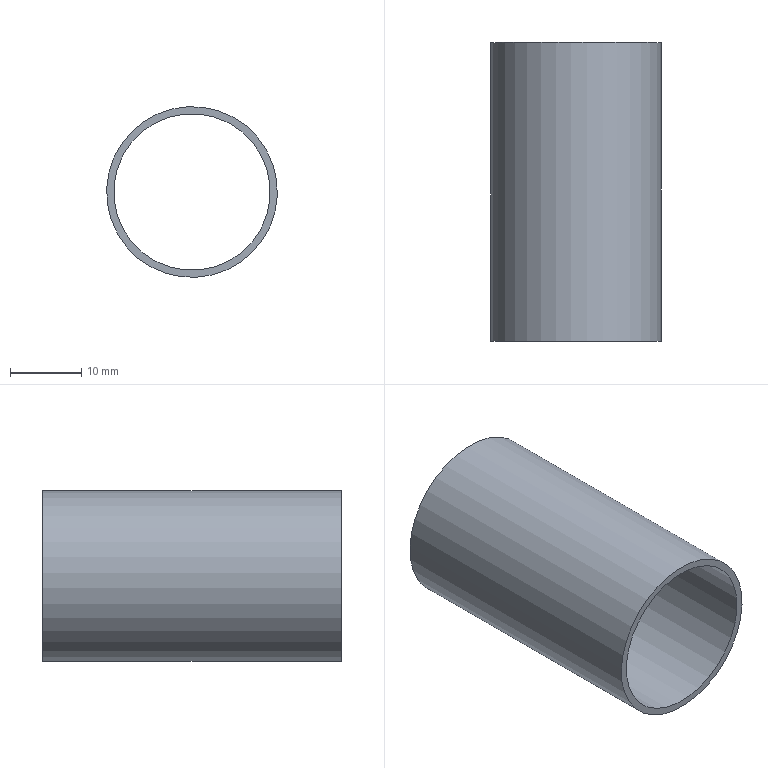Component | NX | ROD_BUSH_UPPER_2 | 1 solid | 4 faces | box 24 x 42 x 24 mm | volume 3035 mm3 | cylinder 2 | plane 2 | commonest cylinder face diameters 24 x1 22 x1
STEP:
#1=CARTESIAN_POINT('',(0.,0.,0.));
#2=DIRECTION('',(0.,0.,1.));
#3=DIRECTION('',(1.,0.,0.));
#4=AXIS2_PLACEMENT_3D('',#1,#2,#3);
#5=CARTESIAN_POINT('',(-172.125,-21.,139.454));
#6=VERTEX_POINT('',#5);
#7=CARTESIAN_POINT('',(-181.305,-21.,131.726));
#8=DIRECTION('',(0.,-1.,0.));
#9=DIRECTION('',(0.765,0.,0.644));
#10=AXIS2_PLACEMENT_3D('',#7,#8,#9);
#11=CIRCLE('',#10,12.);
#12=CARTESIAN_POINT('',(-181.305,-21.,131.726));
#13=DIRECTION('',(0.,1.,0.));
#14=DIRECTION('',(-0.765,0.,-0.644));
#15=AXIS2_PLACEMENT_3D('',#12,#13,#14);
#16=CYLINDRICAL_SURFACE('',#15,12.);
#17=CARTESIAN_POINT('',(9.425,0.));
#18=DIRECTION('',(-1.,0.));
#19=VECTOR('',#18,1.);
#20=LINE('',#17,#19);
#21=(GEOMETRIC_REPRESENTATION_CONTEXT(2)PARAMETRIC_REPRESENTATION_CONTEXT()REPRESENTATION_CONTEXT('',''));
#22=DEFINITIONAL_REPRESENTATION('',(#20),#21);
#23=PCURVE('',#16,#22);
#24=CARTESIAN_POINT('',(-181.305,-21.,131.726));
#25=DIRECTION('',(0.,-1.,0.));
#26=DIRECTION('',(0.765,0.,0.644));
#27=AXIS2_PLACEMENT_3D('',#24,#25,#26);
#28=PLANE('',#27);
#29=CARTESIAN_POINT('',(0.,0.));
#30=DIRECTION('',(1.,0.));
#31=AXIS2_PLACEMENT_2D('',#29,#30);
#32=CIRCLE('',#31,12.);
#33=(GEOMETRIC_REPRESENTATION_CONTEXT(2)PARAMETRIC_REPRESENTATION_CONTEXT()REPRESENTATION_CONTEXT('',''));
#34=DEFINITIONAL_REPRESENTATION('',(#32),#33);
#35=PCURVE('',#28,#34);
#36=SURFACE_CURVE('',#11,(#23,#35),.PCURVE_S1.);
#37=EDGE_CURVE('',#6,#6,#36,.T.);
#38=ORIENTED_EDGE('',*,*,#37,.F.);
#39=CARTESIAN_POINT('',(-172.125,21.,139.454));
#40=VERTEX_POINT('',#39);
#41=CARTESIAN_POINT('',(-172.125,-21.,139.454));
#42=CARTESIAN_POINT('',(-172.125,21.,139.454));
#43=B_SPLINE_CURVE_WITH_KNOTS('',1,(#41,#42),.UNSPECIFIED.,.F.,.F.,(2,2),(0.,42.),.PIECEWISE_BEZIER_KNOTS.);
#44=CARTESIAN_POINT('',(9.425,0.));
#45=DIRECTION('',(0.,1.));
#46=VECTOR('',#45,1.);
#47=LINE('',#44,#46);
#48=(GEOMETRIC_REPRESENTATION_CONTEXT(2)PARAMETRIC_REPRESENTATION_CONTEXT()REPRESENTATION_CONTEXT('',''));
#49=DEFINITIONAL_REPRESENTATION('',(#47),#48);
#50=PCURVE('',#16,#49);
#51=CARTESIAN_POINT('',(3.142,0.));
#52=DIRECTION('',(0.,1.));
#53=VECTOR('',#52,1.);
#54=LINE('',#51,#53);
#55=(GEOMETRIC_REPRESENTATION_CONTEXT(2)PARAMETRIC_REPRESENTATION_CONTEXT()REPRESENTATION_CONTEXT('',''));
#56=DEFINITIONAL_REPRESENTATION('',(#54),#55);
#57=PCURVE('',#16,#56);
#58=SEAM_CURVE('',#43,(#50,#57),.PCURVE_S1.);
#59=EDGE_CURVE('',#6,#40,#58,.T.);
#60=ORIENTED_EDGE('',*,*,#59,.T.);
#61=CARTESIAN_POINT('',(-181.305,21.,131.726));
#62=DIRECTION('',(0.,-1.,0.));
#63=DIRECTION('',(0.765,0.,0.644));
#64=AXIS2_PLACEMENT_3D('',#61,#62,#63);
#65=CIRCLE('',#64,12.);
#66=CARTESIAN_POINT('',(9.425,42.));
#67=DIRECTION('',(-1.,0.));
#68=VECTOR('',#67,1.);
#69=LINE('',#66,#68);
#70=(GEOMETRIC_REPRESENTATION_CONTEXT(2)PARAMETRIC_REPRESENTATION_CONTEXT()REPRESENTATION_CONTEXT('',''));
#71=DEFINITIONAL_REPRESENTATION('',(#69),#70);
#72=PCURVE('',#16,#71);
#73=CARTESIAN_POINT('',(-181.305,21.,131.726));
#74=DIRECTION('',(0.,-1.,0.));
#75=DIRECTION('',(0.765,0.,0.644));
#76=AXIS2_PLACEMENT_3D('',#73,#74,#75);
#77=PLANE('',#76);
#78=CARTESIAN_POINT('',(0.,0.));
#79=DIRECTION('',(1.,0.));
#80=AXIS2_PLACEMENT_2D('',#78,#79);
#81=CIRCLE('',#80,12.);
#82=(GEOMETRIC_REPRESENTATION_CONTEXT(2)PARAMETRIC_REPRESENTATION_CONTEXT()REPRESENTATION_CONTEXT('',''));
#83=DEFINITIONAL_REPRESENTATION('',(#81),#82);
#84=PCURVE('',#77,#83);
#85=SURFACE_CURVE('',#65,(#72,#84),.PCURVE_S1.);
#86=EDGE_CURVE('',#40,#40,#85,.T.);
#87=ORIENTED_EDGE('',*,*,#86,.T.);
#88=ORIENTED_EDGE('',*,*,#59,.F.);
#89=EDGE_LOOP('',(#38,#60,#87,#88));
#90=FACE_BOUND('',#89,.T.);
#91=ADVANCED_FACE('',(#90),#16,.T.);
#92=CARTESIAN_POINT('',(-172.89,-21.,138.81));
#93=VERTEX_POINT('',#92);
#94=CARTESIAN_POINT('',(-181.305,-21.,131.726));
#95=DIRECTION('',(0.,-1.,0.));
#96=DIRECTION('',(0.765,0.,0.644));
#97=AXIS2_PLACEMENT_3D('',#94,#95,#96);
#98=CIRCLE('',#97,11.);
#99=CARTESIAN_POINT('',(-181.305,-21.,131.726));
#100=DIRECTION('',(0.,1.,0.));
#101=DIRECTION('',(-0.765,0.,-0.644));
#102=AXIS2_PLACEMENT_3D('',#99,#100,#101);
#103=CYLINDRICAL_SURFACE('',#102,11.);
#104=CARTESIAN_POINT('',(9.425,0.));
#105=DIRECTION('',(-1.,0.));
#106=VECTOR('',#105,1.);
#107=LINE('',#104,#106);
#108=(GEOMETRIC_REPRESENTATION_CONTEXT(2)PARAMETRIC_REPRESENTATION_CONTEXT()REPRESENTATION_CONTEXT('',''));
#109=DEFINITIONAL_REPRESENTATION('',(#107),#108);
#110=PCURVE('',#103,#109);
#111=CARTESIAN_POINT('',(0.,0.));
#112=DIRECTION('',(1.,-0.));
#113=AXIS2_PLACEMENT_2D('',#111,#112);
#114=CIRCLE('',#113,11.);
#115=(GEOMETRIC_REPRESENTATION_CONTEXT(2)PARAMETRIC_REPRESENTATION_CONTEXT()REPRESENTATION_CONTEXT('',''));
#116=DEFINITIONAL_REPRESENTATION('',(#114),#115);
#117=PCURVE('',#28,#116);
#118=SURFACE_CURVE('',#98,(#110,#117),.PCURVE_S1.);
#119=EDGE_CURVE('',#93,#93,#118,.T.);
#120=ORIENTED_EDGE('',*,*,#119,.F.);
#121=CARTESIAN_POINT('',(-172.89,21.,138.81));
#122=VERTEX_POINT('',#121);
#123=CARTESIAN_POINT('',(-172.89,-21.,138.81));
#124=CARTESIAN_POINT('',(-172.89,21.,138.81));
#125=B_SPLINE_CURVE_WITH_KNOTS('',1,(#123,#124),.UNSPECIFIED.,.F.,.F.,(2,2),(0.,42.),.PIECEWISE_BEZIER_KNOTS.);
#126=CARTESIAN_POINT('',(9.425,0.));
#127=DIRECTION('',(0.,1.));
#128=VECTOR('',#127,1.);
#129=LINE('',#126,#128);
#130=(GEOMETRIC_REPRESENTATION_CONTEXT(2)PARAMETRIC_REPRESENTATION_CONTEXT()REPRESENTATION_CONTEXT('',''));
#131=DEFINITIONAL_REPRESENTATION('',(#129),#130);
#132=PCURVE('',#103,#131);
#133=CARTESIAN_POINT('',(3.142,0.));
#134=DIRECTION('',(0.,1.));
#135=VECTOR('',#134,1.);
#136=LINE('',#133,#135);
#137=(GEOMETRIC_REPRESENTATION_CONTEXT(2)PARAMETRIC_REPRESENTATION_CONTEXT()REPRESENTATION_CONTEXT('',''));
#138=DEFINITIONAL_REPRESENTATION('',(#136),#137);
#139=PCURVE('',#103,#138);
#140=SEAM_CURVE('',#125,(#132,#139),.PCURVE_S1.);
#141=EDGE_CURVE('',#93,#122,#140,.T.);
#142=ORIENTED_EDGE('',*,*,#141,.T.);
#143=CARTESIAN_POINT('',(-181.305,21.,131.726));
#144=DIRECTION('',(0.,-1.,0.));
#145=DIRECTION('',(0.765,0.,0.644));
#146=AXIS2_PLACEMENT_3D('',#143,#144,#145);
#147=CIRCLE('',#146,11.);
#148=CARTESIAN_POINT('',(9.425,42.));
#149=DIRECTION('',(-1.,0.));
#150=VECTOR('',#149,1.);
#151=LINE('',#148,#150);
#152=(GEOMETRIC_REPRESENTATION_CONTEXT(2)PARAMETRIC_REPRESENTATION_CONTEXT()REPRESENTATION_CONTEXT('',''));
#153=DEFINITIONAL_REPRESENTATION('',(#151),#152);
#154=PCURVE('',#103,#153);
#155=CARTESIAN_POINT('',(0.,0.));
#156=DIRECTION('',(1.,-0.));
#157=AXIS2_PLACEMENT_2D('',#155,#156);
#158=CIRCLE('',#157,11.);
#159=(GEOMETRIC_REPRESENTATION_CONTEXT(2)PARAMETRIC_REPRESENTATION_CONTEXT()REPRESENTATION_CONTEXT('',''));
#160=DEFINITIONAL_REPRESENTATION('',(#158),#159);
#161=PCURVE('',#77,#160);
#162=SURFACE_CURVE('',#147,(#154,#161),.PCURVE_S1.);
#163=EDGE_CURVE('',#122,#122,#162,.T.);
#164=ORIENTED_EDGE('',*,*,#163,.T.);
#165=ORIENTED_EDGE('',*,*,#141,.F.);
#166=EDGE_LOOP('',(#120,#142,#164,#165));
#167=FACE_BOUND('',#166,.F.);
#168=ADVANCED_FACE('',(#167),#103,.F.);
#169=ORIENTED_EDGE('',*,*,#37,.T.);
#170=EDGE_LOOP('',(#169));
#171=FACE_BOUND('',#170,.T.);
#172=ORIENTED_EDGE('',*,*,#119,.F.);
#173=EDGE_LOOP('',(#172));
#174=FACE_BOUND('',#173,.T.);
#175=ADVANCED_FACE('',(#171,#174),#28,.T.);
#176=ORIENTED_EDGE('',*,*,#86,.F.);
#177=EDGE_LOOP('',(#176));
#178=FACE_BOUND('',#177,.T.);
#179=ORIENTED_EDGE('',*,*,#163,.T.);
#180=EDGE_LOOP('',(#179));
#181=FACE_BOUND('',#180,.T.);
#182=ADVANCED_FACE('',(#178,#181),#77,.F.);
#183=CLOSED_SHELL('',(#91,#168,#175,#182));
#184=MANIFOLD_SOLID_BREP('',#183);
#185=(LENGTH_UNIT()NAMED_UNIT(*)SI_UNIT(.MILLI.,.METRE.));
#186=UNCERTAINTY_MEASURE_WITH_UNIT(LENGTH_MEASURE(0.00001),#185,'','');
#187=(NAMED_UNIT(*)PLANE_ANGLE_UNIT()SI_UNIT($,.RADIAN.));
#188=(NAMED_UNIT(*)SI_UNIT($,.STERADIAN.)SOLID_ANGLE_UNIT());
#189=(GEOMETRIC_REPRESENTATION_CONTEXT(3)GLOBAL_UNCERTAINTY_ASSIGNED_CONTEXT((#186))GLOBAL_UNIT_ASSIGNED_CONTEXT((#185,#187,#188))REPRESENTATION_CONTEXT('',''));
#190=ADVANCED_BREP_SHAPE_REPRESENTATION('',(#4,#184),#189);